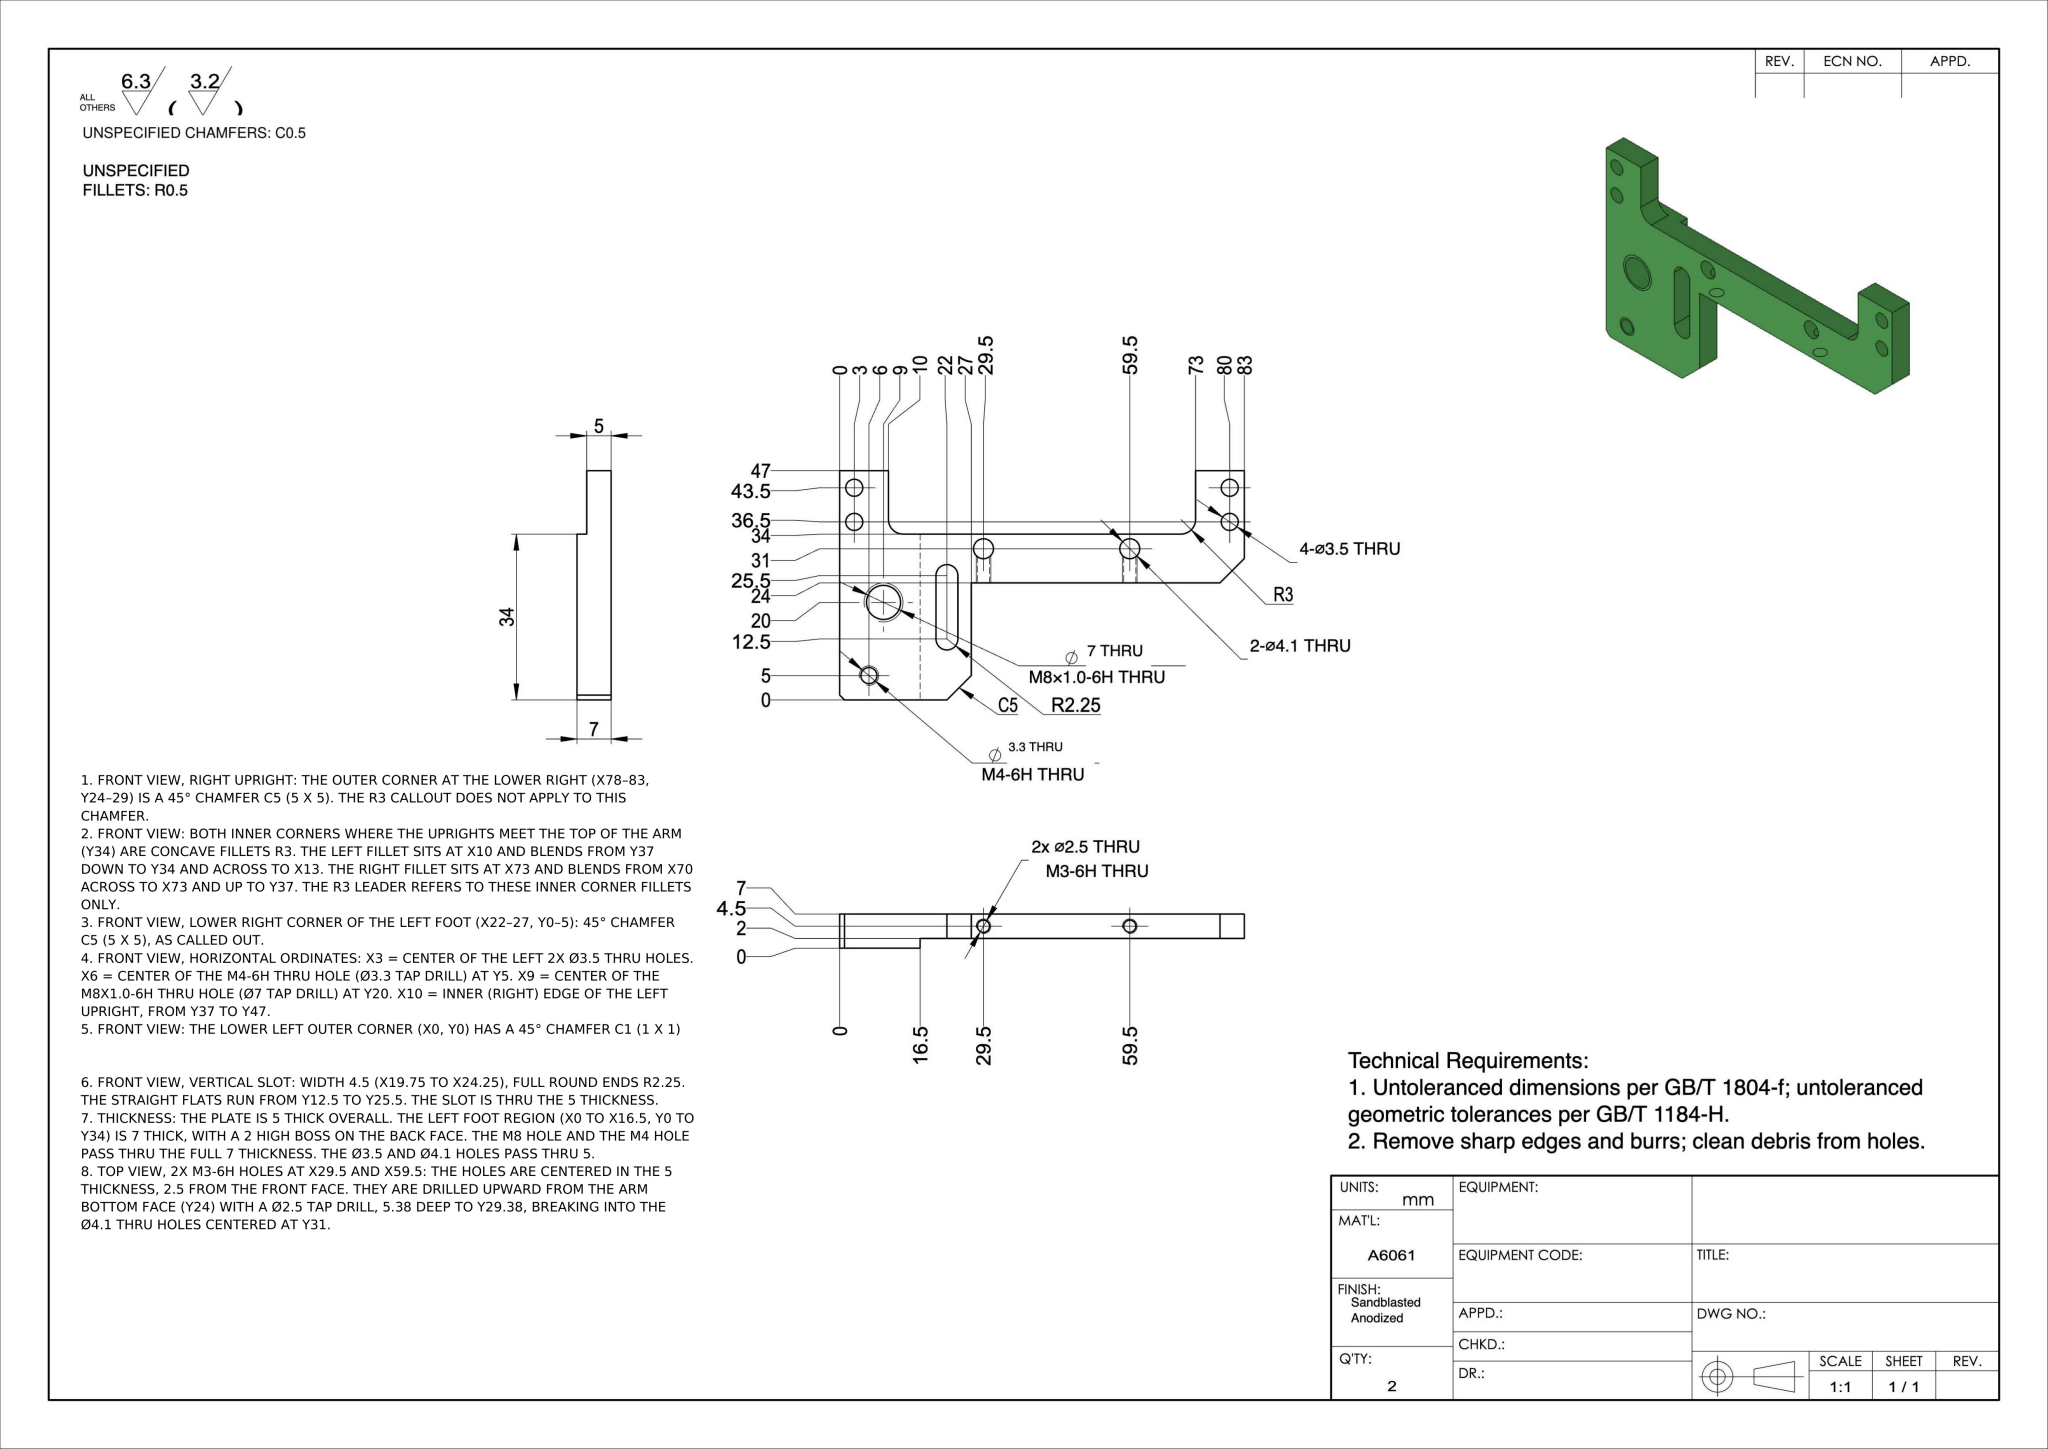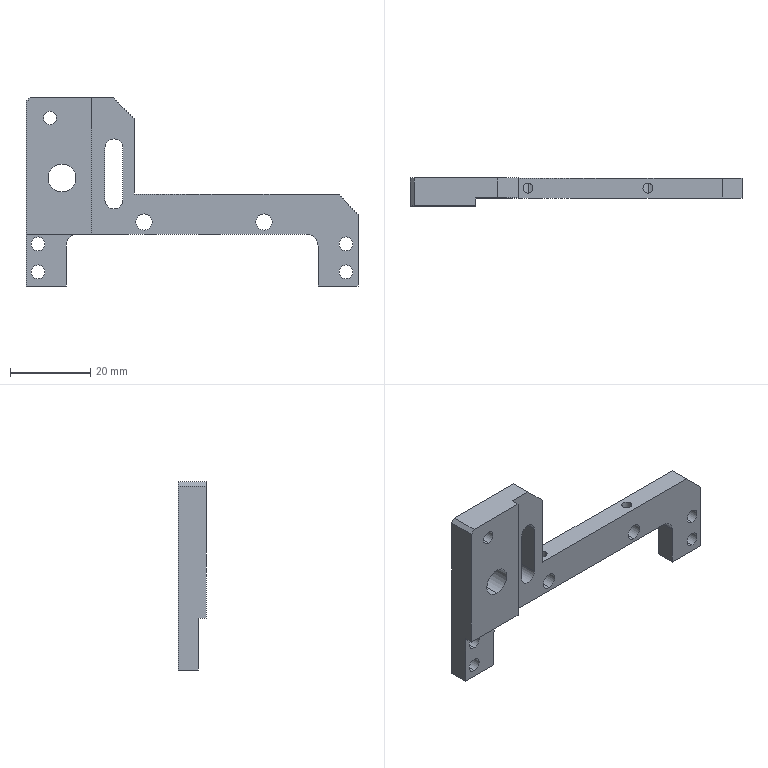Part | NX | mm | Stepped Mounting Bracket | 1 solid | 45 faces | box 83 x 7 x 47 mm | volume 8628 mm3 | cylinder 25 | plane 20 | commonest cylinder face diameters 3.5 x8 2.5 x4 4.1 x4 4.5 x3 7 x2 3.3 x2 6 x2